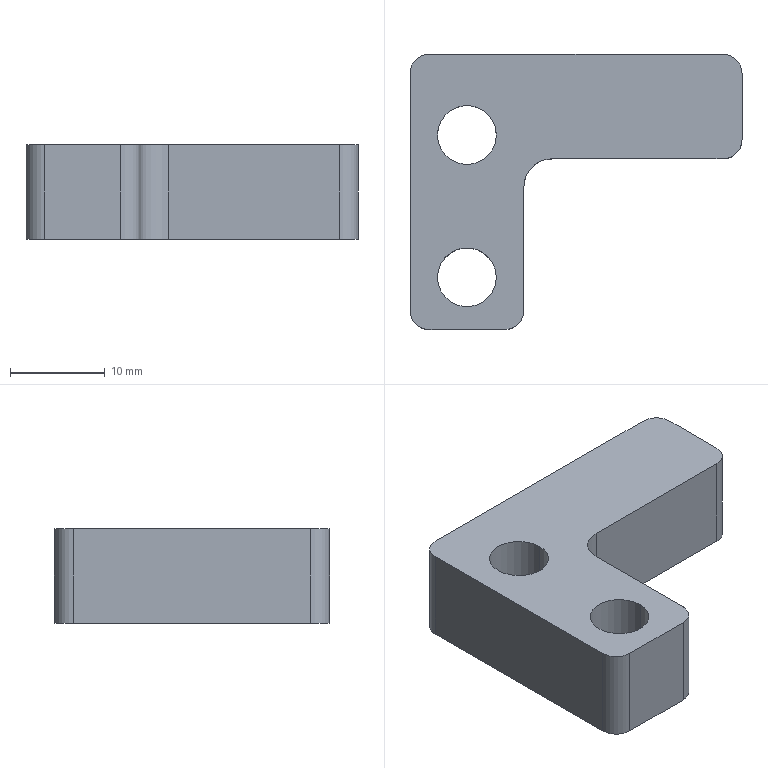CAM job | Mastercam | mm | 8 operations | part box 35 x 29 x 10
1. Facing | 24 - 100 平铣刀
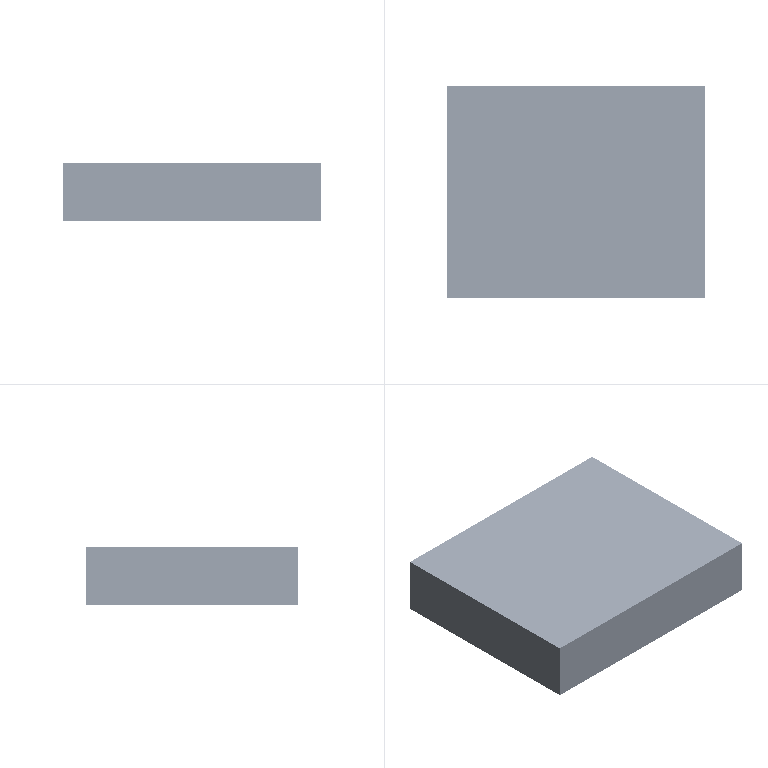2. 2D High Speed (2D Dynamic Mill) | 10 - 10 平铣刀
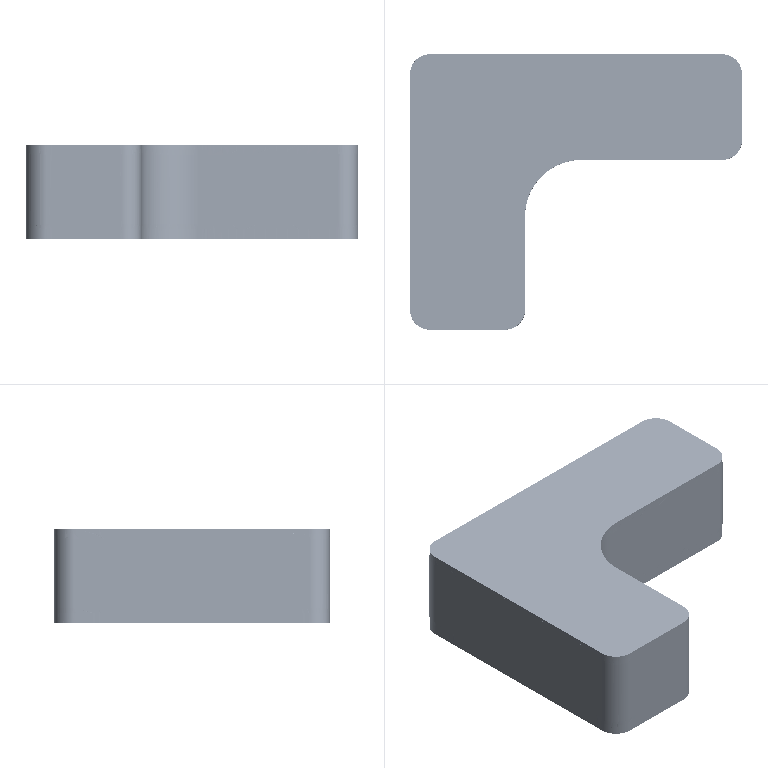3. Contour (Remachining) | 6 - 6 平铣刀
4. Contour (Ramp) | 10 - 10 平铣刀
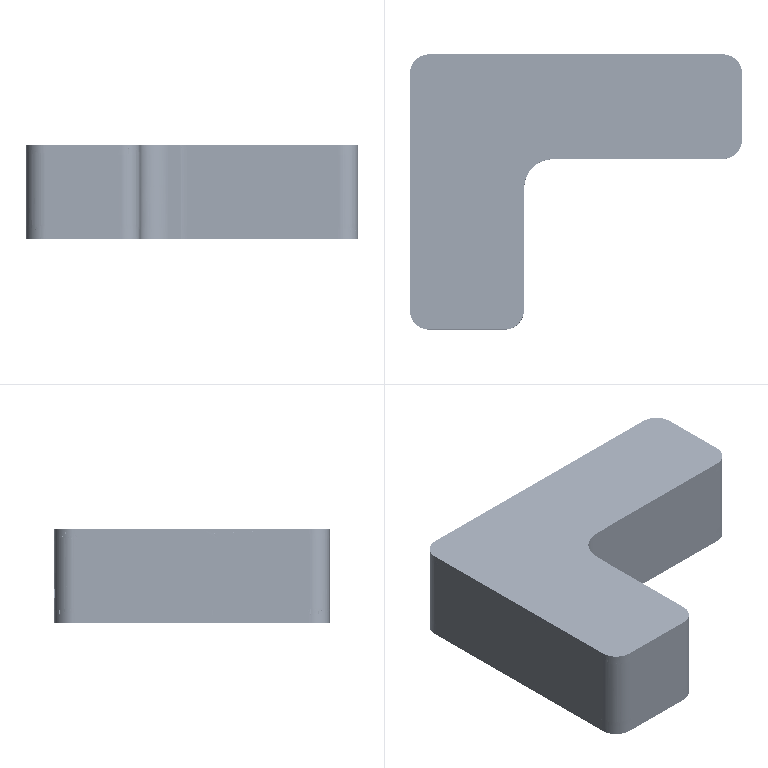5. Drill/Counterbore | 7 - 4 倒角刀
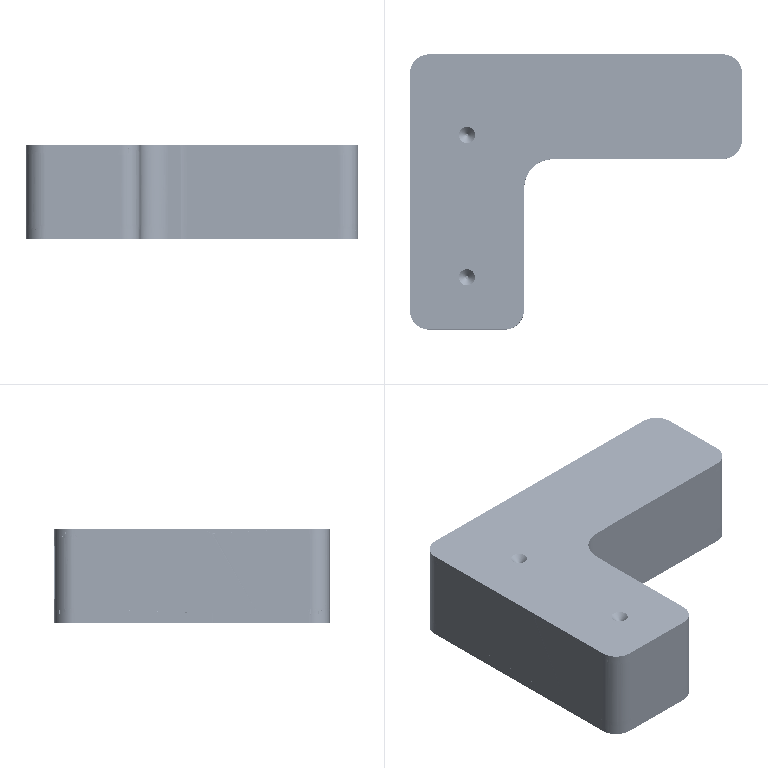6. Contour (2D chamfer) | 7 - 4 倒角刀
7. Facing | 10 - 10 平铣刀
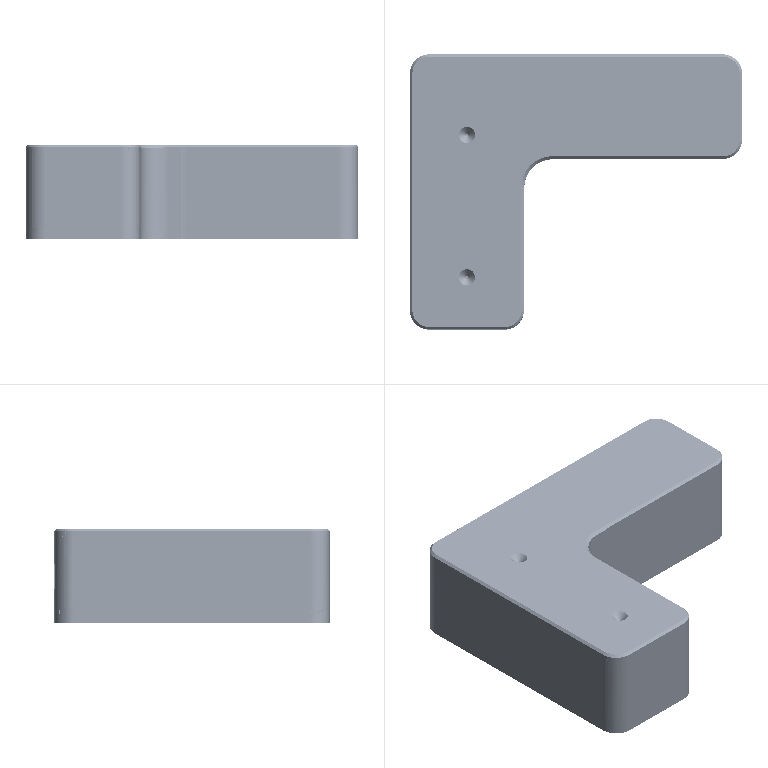8. Contour (2D chamfer) | 7 - 4 倒角刀